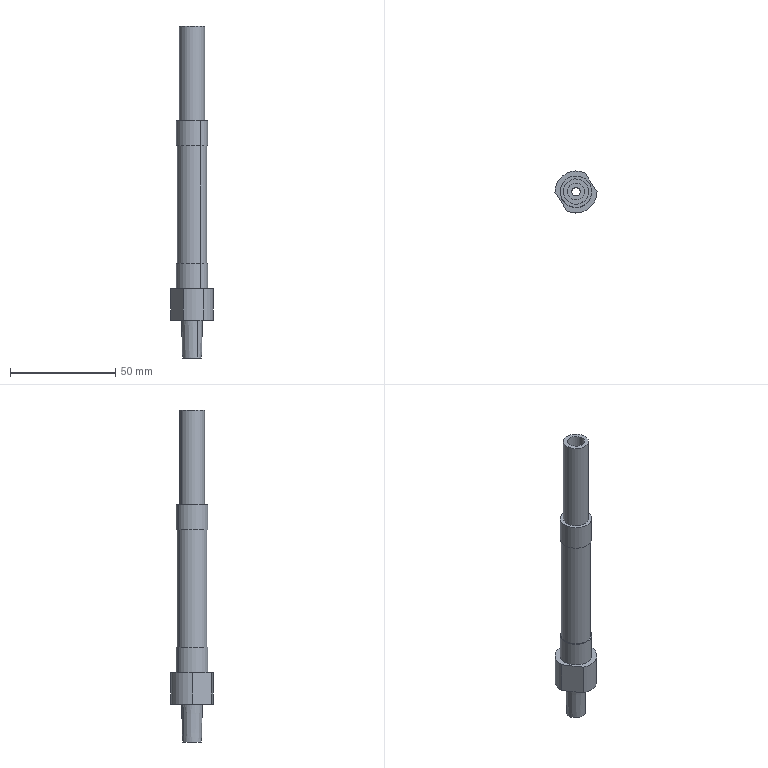Component | SolidWorks | Axis-2 | 1 solid | 27 faces | box 20 x 20 x 158 mm | volume 19937 mm3 | cylinder 15 | plane 10 | cone 2 | commonest cylinder face diameters 15 x4 20 x3 4 x2 8 x2 12 x2 14 x2
build123d program:
from build123d import *

# Parameters (mm, degrees)
SKETCH3_R      = 4
EXTRUDE1_DEPTH = 45
SKETCH4_R      = 2
EXTRUDE2_DEPTH = 159.632
SKETCH5_W      = 1.5
SKETCH5_H      = 15
EXTRUDE3_DEPTH = 10


with BuildPart() as part:
    # Sketch1 → Revolve1 (revolve)
    with BuildSketch(Plane.XY, mode=Mode.PRIVATE) as revolve1_sk:
        Polygon((0, 52.72), (4.5, 52.72), (5, 34.72), (10, 34.72), (10, 19.72), (7.5, 19.72), (7.5, 7.72), (7, 7.72), (7, -48.28), (7.5, -48.28), (7.5, -60.28), (6, -60.28), (6, -105.28), (0, -105.28), align=None)
    revolve(revolve1_sk.sketch.rotate(Axis((0, 0, 0), (0, 1, 0)), 90), axis=Axis((0, 0, 0), (0, 1, 0)))

    # Sketch3 → Extrude1 (cut)
    with BuildSketch(Plane.XZ.offset(105.28)):
        with Locations(Location((0, 0, 0), (0, 0, 270))):
            Circle(SKETCH3_R)
    extrude(amount=-EXTRUDE1_DEPTH, mode=Mode.SUBTRACT)

    # Sketch4 → Extrude2 (cut, through all)
    with BuildSketch(Plane(origin=(0, 52.72, 0), x_dir=(1, 0, 0), z_dir=(0, 1, 0))):
        with Locations(Location((0, 0, 0), (0, 0, 270))):
            Circle(SKETCH4_R)
    extrude(amount=-EXTRUDE2_DEPTH, mode=Mode.SUBTRACT)

    # Sketch5 → Extrude3 (cut, symmetric)
    with BuildSketch(Plane.XY):
        with Locations((9.25, 27.22)):
            Rectangle(SKETCH5_W, SKETCH5_H)
        with Locations((-9.25, 27.22)):
            Rectangle(SKETCH5_W, SKETCH5_H)
    extrude(amount=EXTRUDE3_DEPTH, both=True, mode=Mode.SUBTRACT)


solid = part.part

# Placed as in the assembly
solid = solid.moved(Location((-110.944, 573.983, 177.508), (-90, -33.719, 0)))
STEP:
#1=COLOUR_RGB('',0.7922,0.8196,0.9333);
#2=FILL_AREA_STYLE_COLOUR('',#1);
#3=FILL_AREA_STYLE('',(#2));
#4=SURFACE_STYLE_FILL_AREA(#3);
#5=SURFACE_SIDE_STYLE('',(#4));
#6=SURFACE_STYLE_USAGE(.BOTH.,#5);
#7=PRESENTATION_STYLE_ASSIGNMENT((#6));
#8=CARTESIAN_POINT('',(-4.412,22.663,9.362));
#9=VERTEX_POINT('',#8);
#10=CARTESIAN_POINT('',(-4.324,22.532,9.362));
#11=VERTEX_POINT('',#10);
#12=CARTESIAN_POINT('',(-4.368,22.598,9.362));
#13=DIRECTION('',(0.,0.,1.));
#14=DIRECTION('',(0.5551,-0.8318,0.));
#15=AXIS2_PLACEMENT_3D('',#12,#13,#14);
#16=CIRCLE('',#15,0.07874);
#17=EDGE_CURVE('',#9,#11,#16,.T.);
#18=ORIENTED_EDGE('',*,*,#17,.T.);
#19=CARTESIAN_POINT('',(-4.324,22.532,4.913));
#20=VERTEX_POINT('',#19);
#21=CARTESIAN_POINT('',(-4.324,22.532,11.133));
#22=DIRECTION('',(0.,0.,-1.));
#23=VECTOR('',#22,39.37);
#24=LINE('',#21,#23);
#25=EDGE_CURVE('',#11,#20,#24,.T.);
#26=ORIENTED_EDGE('',*,*,#25,.T.);
#27=CARTESIAN_POINT('',(-4.412,22.663,4.913));
#28=VERTEX_POINT('',#27);
#29=CARTESIAN_POINT('',(-4.368,22.598,4.913));
#30=DIRECTION('',(0.,0.,-1.));
#31=DIRECTION('',(-0.5551,0.8318,0.));
#32=AXIS2_PLACEMENT_3D('',#29,#30,#31);
#33=CIRCLE('',#32,0.07874);
#34=EDGE_CURVE('',#20,#28,#33,.T.);
#35=ORIENTED_EDGE('',*,*,#34,.T.);
#36=CARTESIAN_POINT('',(-4.412,22.663,11.133));
#37=DIRECTION('',(0.,0.,-1.));
#38=VECTOR('',#37,39.37);
#39=LINE('',#36,#38);
#40=EDGE_CURVE('',#9,#28,#39,.T.);
#41=ORIENTED_EDGE('',*,*,#40,.F.);
#42=EDGE_LOOP('',(#18,#26,#35,#41));
#43=FACE_OUTER_BOUND('',#42,.T.);
#44=CARTESIAN_POINT('',(-4.368,22.598,11.133));
#45=DIRECTION('',(0.,0.,-1.));
#46=DIRECTION('',(-0.5551,0.8318,0.));
#47=AXIS2_PLACEMENT_3D('',#44,#45,#46);
#48=CYLINDRICAL_SURFACE('',#47,0.07874);
#49=ADVANCED_FACE('',(#43),#48,.F.);
#50=CARTESIAN_POINT('',(-4.28,22.467,9.362));
#51=VERTEX_POINT('',#50);
#52=CARTESIAN_POINT('',(-4.455,22.729,9.362));
#53=VERTEX_POINT('',#52);
#54=CARTESIAN_POINT('',(-4.368,22.598,9.362));
#55=DIRECTION('',(0.,0.,-1.));
#56=DIRECTION('',(0.5551,-0.8318,0.));
#57=AXIS2_PLACEMENT_3D('',#54,#55,#56);
#58=CIRCLE('',#57,0.1575);
#59=EDGE_CURVE('',#51,#53,#58,.T.);
#60=ORIENTED_EDGE('',*,*,#59,.T.);
#61=CARTESIAN_POINT('',(-4.455,22.729,11.133));
#62=VERTEX_POINT('',#61);
#63=CARTESIAN_POINT('',(-4.455,22.729,8.916));
#64=DIRECTION('',(0.,0.,1.));
#65=VECTOR('',#64,39.37);
#66=LINE('',#63,#65);
#67=EDGE_CURVE('',#53,#62,#66,.T.);
#68=ORIENTED_EDGE('',*,*,#67,.T.);
#69=CARTESIAN_POINT('',(-4.28,22.467,11.133));
#70=VERTEX_POINT('',#69);
#71=CARTESIAN_POINT('',(-4.368,22.598,11.133));
#72=DIRECTION('',(0.,0.,1.));
#73=DIRECTION('',(0.5551,-0.8318,0.));
#74=AXIS2_PLACEMENT_3D('',#71,#72,#73);
#75=CIRCLE('',#74,0.1575);
#76=EDGE_CURVE('',#62,#70,#75,.T.);
#77=ORIENTED_EDGE('',*,*,#76,.T.);
#78=CARTESIAN_POINT('',(-4.28,22.467,8.916));
#79=DIRECTION('',(0.,0.,1.));
#80=VECTOR('',#79,39.37);
#81=LINE('',#78,#80);
#82=EDGE_CURVE('',#51,#70,#81,.T.);
#83=ORIENTED_EDGE('',*,*,#82,.F.);
#84=EDGE_LOOP('',(#60,#68,#77,#83));
#85=FACE_OUTER_BOUND('',#84,.T.);
#86=CARTESIAN_POINT('',(-4.368,22.598,8.916));
#87=DIRECTION('',(0.,0.,1.));
#88=DIRECTION('',(0.5551,-0.8318,0.));
#89=AXIS2_PLACEMENT_3D('',#86,#87,#88);
#90=CYLINDRICAL_SURFACE('',#89,0.1575);
#91=ADVANCED_FACE('',(#85),#90,.F.);
#92=CARTESIAN_POINT('',(-4.237,22.401,9.362));
#93=VERTEX_POINT('',#92);
#94=CARTESIAN_POINT('',(-4.499,22.794,9.362));
#95=VERTEX_POINT('',#94);
#96=CARTESIAN_POINT('',(-4.368,22.598,9.362));
#97=DIRECTION('',(0.,0.,1.));
#98=DIRECTION('',(0.5551,-0.8318,0.));
#99=AXIS2_PLACEMENT_3D('',#96,#97,#98);
#100=CIRCLE('',#99,0.2362);
#101=EDGE_CURVE('',#93,#95,#100,.T.);
#102=ORIENTED_EDGE('',*,*,#101,.T.);
#103=CARTESIAN_POINT('',(-4.499,22.794,11.133));
#104=VERTEX_POINT('',#103);
#105=CARTESIAN_POINT('',(-4.499,22.794,6.989));
#106=DIRECTION('',(0.,0.,1.));
#107=VECTOR('',#106,39.37);
#108=LINE('',#105,#107);
#109=EDGE_CURVE('',#95,#104,#108,.T.);
#110=ORIENTED_EDGE('',*,*,#109,.T.);
#111=CARTESIAN_POINT('',(-4.237,22.401,11.133));
#112=VERTEX_POINT('',#111);
#113=CARTESIAN_POINT('',(-4.368,22.598,11.133));
#114=DIRECTION('',(0.,0.,1.));
#115=DIRECTION('',(0.5551,-0.8318,0.));
#116=AXIS2_PLACEMENT_3D('',#113,#114,#115);
#117=CIRCLE('',#116,0.2362);
#118=EDGE_CURVE('',#112,#104,#117,.T.);
#119=ORIENTED_EDGE('',*,*,#118,.F.);
#120=CARTESIAN_POINT('',(-4.237,22.401,6.989));
#121=DIRECTION('',(0.,0.,1.));
#122=VECTOR('',#121,39.37);
#123=LINE('',#120,#122);
#124=EDGE_CURVE('',#93,#112,#123,.T.);
#125=ORIENTED_EDGE('',*,*,#124,.F.);
#126=EDGE_LOOP('',(#102,#110,#119,#125));
#127=FACE_OUTER_BOUND('',#126,.T.);
#128=CARTESIAN_POINT('',(-4.368,22.598,6.989));
#129=DIRECTION('',(0.,0.,1.));
#130=DIRECTION('',(0.5551,-0.8318,0.));
#131=AXIS2_PLACEMENT_3D('',#128,#129,#130);
#132=CYLINDRICAL_SURFACE('',#131,0.2362);
#133=ADVANCED_FACE('',(#127),#132,.T.);
#134=CARTESIAN_POINT('',(-4.204,22.352,8.889));
#135=VERTEX_POINT('',#134);
#136=CARTESIAN_POINT('',(-4.532,22.843,8.889));
#137=VERTEX_POINT('',#136);
#138=CARTESIAN_POINT('',(-4.368,22.598,8.889));
#139=DIRECTION('',(0.,0.,1.));
#140=DIRECTION('',(0.5551,-0.8318,0.));
#141=AXIS2_PLACEMENT_3D('',#138,#139,#140);
#142=CIRCLE('',#141,0.2953);
#143=EDGE_CURVE('',#135,#137,#142,.T.);
#144=ORIENTED_EDGE('',*,*,#143,.T.);
#145=CARTESIAN_POINT('',(-4.532,22.843,9.362));
#146=VERTEX_POINT('',#145);
#147=CARTESIAN_POINT('',(-4.532,22.843,6.989));
#148=DIRECTION('',(0.,0.,1.));
#149=VECTOR('',#148,39.37);
#150=LINE('',#147,#149);
#151=EDGE_CURVE('',#137,#146,#150,.T.);
#152=ORIENTED_EDGE('',*,*,#151,.T.);
#153=CARTESIAN_POINT('',(-4.204,22.352,9.362));
#154=VERTEX_POINT('',#153);
#155=CARTESIAN_POINT('',(-4.368,22.598,9.362));
#156=DIRECTION('',(0.,0.,1.));
#157=DIRECTION('',(0.5551,-0.8318,0.));
#158=AXIS2_PLACEMENT_3D('',#155,#156,#157);
#159=CIRCLE('',#158,0.2953);
#160=EDGE_CURVE('',#154,#146,#159,.T.);
#161=ORIENTED_EDGE('',*,*,#160,.F.);
#162=CARTESIAN_POINT('',(-4.204,22.352,6.989));
#163=DIRECTION('',(0.,0.,1.));
#164=VECTOR('',#163,39.37);
#165=LINE('',#162,#164);
#166=EDGE_CURVE('',#135,#154,#165,.T.);
#167=ORIENTED_EDGE('',*,*,#166,.F.);
#168=EDGE_LOOP('',(#144,#152,#161,#167));
#169=FACE_OUTER_BOUND('',#168,.T.);
#170=CARTESIAN_POINT('',(-4.368,22.598,6.989));
#171=DIRECTION('',(0.,0.,1.));
#172=DIRECTION('',(0.5551,-0.8318,0.));
#173=AXIS2_PLACEMENT_3D('',#170,#171,#172);
#174=CYLINDRICAL_SURFACE('',#173,0.2953);
#175=ADVANCED_FACE('',(#169),#174,.T.);
#176=CARTESIAN_POINT('',(-4.215,22.369,6.685));
#177=VERTEX_POINT('',#176);
#178=CARTESIAN_POINT('',(-4.521,22.827,6.685));
#179=VERTEX_POINT('',#178);
#180=CARTESIAN_POINT('',(-4.368,22.598,6.685));
#181=DIRECTION('',(0.,0.,1.));
#182=DIRECTION('',(0.5551,-0.8318,0.));
#183=AXIS2_PLACEMENT_3D('',#180,#181,#182);
#184=CIRCLE('',#183,0.2756);
#185=EDGE_CURVE('',#177,#179,#184,.T.);
#186=ORIENTED_EDGE('',*,*,#185,.T.);
#187=CARTESIAN_POINT('',(-4.521,22.827,8.889));
#188=VERTEX_POINT('',#187);
#189=CARTESIAN_POINT('',(-4.521,22.827,6.989));
#190=DIRECTION('',(0.,0.,1.));
#191=VECTOR('',#190,39.37);
#192=LINE('',#189,#191);
#193=EDGE_CURVE('',#179,#188,#192,.T.);
#194=ORIENTED_EDGE('',*,*,#193,.T.);
#195=CARTESIAN_POINT('',(-4.215,22.369,8.889));
#196=VERTEX_POINT('',#195);
#197=CARTESIAN_POINT('',(-4.368,22.598,8.889));
#198=DIRECTION('',(0.,0.,1.));
#199=DIRECTION('',(0.5551,-0.8318,0.));
#200=AXIS2_PLACEMENT_3D('',#197,#198,#199);
#201=CIRCLE('',#200,0.2756);
#202=EDGE_CURVE('',#196,#188,#201,.T.);
#203=ORIENTED_EDGE('',*,*,#202,.F.);
#204=CARTESIAN_POINT('',(-4.215,22.369,6.989));
#205=DIRECTION('',(0.,0.,1.));
#206=VECTOR('',#205,39.37);
#207=LINE('',#204,#206);
#208=EDGE_CURVE('',#177,#196,#207,.T.);
#209=ORIENTED_EDGE('',*,*,#208,.F.);
#210=EDGE_LOOP('',(#186,#194,#203,#209));
#211=FACE_OUTER_BOUND('',#210,.T.);
#212=CARTESIAN_POINT('',(-4.368,22.598,6.989));
#213=DIRECTION('',(0.,0.,1.));
#214=DIRECTION('',(0.5551,-0.8318,0.));
#215=AXIS2_PLACEMENT_3D('',#212,#213,#214);
#216=CYLINDRICAL_SURFACE('',#215,0.2756);
#217=ADVANCED_FACE('',(#211),#216,.T.);
#218=CARTESIAN_POINT('',(-4.204,22.352,6.212));
#219=VERTEX_POINT('',#218);
#220=CARTESIAN_POINT('',(-4.532,22.843,6.212));
#221=VERTEX_POINT('',#220);
#222=CARTESIAN_POINT('',(-4.368,22.598,6.212));
#223=DIRECTION('',(0.,0.,1.));
#224=DIRECTION('',(0.5551,-0.8318,0.));
#225=AXIS2_PLACEMENT_3D('',#222,#223,#224);
#226=CIRCLE('',#225,0.2953);
#227=EDGE_CURVE('',#219,#221,#226,.T.);
#228=ORIENTED_EDGE('',*,*,#227,.T.);
#229=CARTESIAN_POINT('',(-4.532,22.843,6.685));
#230=VERTEX_POINT('',#229);
#231=CARTESIAN_POINT('',(-4.532,22.843,6.989));
#232=DIRECTION('',(0.,0.,1.));
#233=VECTOR('',#232,39.37);
#234=LINE('',#231,#233);
#235=EDGE_CURVE('',#221,#230,#234,.T.);
#236=ORIENTED_EDGE('',*,*,#235,.T.);
#237=CARTESIAN_POINT('',(-4.204,22.352,6.685));
#238=VERTEX_POINT('',#237);
#239=CARTESIAN_POINT('',(-4.368,22.598,6.685));
#240=DIRECTION('',(0.,0.,1.));
#241=DIRECTION('',(0.5551,-0.8318,0.));
#242=AXIS2_PLACEMENT_3D('',#239,#240,#241);
#243=CIRCLE('',#242,0.2953);
#244=EDGE_CURVE('',#238,#230,#243,.T.);
#245=ORIENTED_EDGE('',*,*,#244,.F.);
#246=CARTESIAN_POINT('',(-4.204,22.352,6.989));
#247=DIRECTION('',(0.,0.,1.));
#248=VECTOR('',#247,39.37);
#249=LINE('',#246,#248);
#250=EDGE_CURVE('',#219,#238,#249,.T.);
#251=ORIENTED_EDGE('',*,*,#250,.F.);
#252=EDGE_LOOP('',(#228,#236,#245,#251));
#253=FACE_OUTER_BOUND('',#252,.T.);
#254=CARTESIAN_POINT('',(-4.368,22.598,6.989));
#255=DIRECTION('',(0.,0.,1.));
#256=DIRECTION('',(0.5551,-0.8318,0.));
#257=AXIS2_PLACEMENT_3D('',#254,#255,#256);
#258=CYLINDRICAL_SURFACE('',#257,0.2953);
#259=ADVANCED_FACE('',(#253),#258,.T.);
#260=CARTESIAN_POINT('',(-4.531,22.239,5.622));
#261=VERTEX_POINT('',#260);
#262=CARTESIAN_POINT('',(-4.149,22.27,5.622));
#263=VERTEX_POINT('',#262);
#264=CARTESIAN_POINT('',(-4.368,22.598,5.622));
#265=DIRECTION('',(0.,0.,1.));
#266=DIRECTION('',(0.5551,-0.8318,0.));
#267=AXIS2_PLACEMENT_3D('',#264,#265,#266);
#268=CIRCLE('',#267,0.3937);
#269=EDGE_CURVE('',#261,#263,#268,.T.);
#270=ORIENTED_EDGE('',*,*,#269,.T.);
#271=CARTESIAN_POINT('',(-4.149,22.27,6.212));
#272=VERTEX_POINT('',#271);
#273=CARTESIAN_POINT('',(-4.149,22.27,6.989));
#274=DIRECTION('',(0.,0.,1.));
#275=VECTOR('',#274,39.37);
#276=LINE('',#273,#275);
#277=EDGE_CURVE('',#263,#272,#276,.T.);
#278=ORIENTED_EDGE('',*,*,#277,.T.);
#279=CARTESIAN_POINT('',(-4.531,22.239,6.212));
#280=VERTEX_POINT('',#279);
#281=CARTESIAN_POINT('',(-4.368,22.598,6.212));
#282=DIRECTION('',(0.,0.,1.));
#283=DIRECTION('',(0.5551,-0.8318,0.));
#284=AXIS2_PLACEMENT_3D('',#281,#282,#283);
#285=CIRCLE('',#284,0.3937);
#286=EDGE_CURVE('',#280,#272,#285,.T.);
#287=ORIENTED_EDGE('',*,*,#286,.F.);
#288=CARTESIAN_POINT('',(-4.531,22.239,6.989));
#289=DIRECTION('',(0.,0.,1.));
#290=VECTOR('',#289,39.37);
#291=LINE('',#288,#290);
#292=EDGE_CURVE('',#261,#280,#291,.T.);
#293=ORIENTED_EDGE('',*,*,#292,.F.);
#294=EDGE_LOOP('',(#270,#278,#287,#293));
#295=FACE_OUTER_BOUND('',#294,.T.);
#296=CARTESIAN_POINT('',(-4.368,22.598,6.989));
#297=DIRECTION('',(0.,0.,1.));
#298=DIRECTION('',(0.5551,-0.8318,0.));
#299=AXIS2_PLACEMENT_3D('',#296,#297,#298);
#300=CYLINDRICAL_SURFACE('',#299,0.3937);
#301=ADVANCED_FACE('',(#295),#300,.T.);
#302=CARTESIAN_POINT('',(-4.27,22.45,4.913));
#303=VERTEX_POINT('',#302);
#304=CARTESIAN_POINT('',(-4.466,22.745,4.913));
#305=VERTEX_POINT('',#304);
#306=CARTESIAN_POINT('',(-4.368,22.598,4.913));
#307=DIRECTION('',(0.,0.,1.));
#308=DIRECTION('',(0.5551,-0.8318,0.));
#309=AXIS2_PLACEMENT_3D('',#306,#307,#308);
#310=CIRCLE('',#309,0.1772);
#311=EDGE_CURVE('',#303,#305,#310,.T.);
#312=ORIENTED_EDGE('',*,*,#311,.T.);
#313=CARTESIAN_POINT('',(-4.477,22.762,5.622));
#314=VERTEX_POINT('',#313);
#315=CARTESIAN_POINT('',(-4.477,22.762,5.622));
#316=DIRECTION('',(-0.01541,0.0231,0.9996));
#317=VECTOR('',#316,39.37);
#318=LINE('',#315,#317);
#319=EDGE_CURVE('',#305,#314,#318,.T.);
#320=ORIENTED_EDGE('',*,*,#319,.T.);
#321=CARTESIAN_POINT('',(-4.259,22.434,5.622));
#322=VERTEX_POINT('',#321);
#323=CARTESIAN_POINT('',(-4.368,22.598,5.622));
#324=DIRECTION('',(0.,0.,1.));
#325=DIRECTION('',(0.5551,-0.8318,0.));
#326=AXIS2_PLACEMENT_3D('',#323,#324,#325);
#327=CIRCLE('',#326,0.1969);
#328=EDGE_CURVE('',#322,#314,#327,.T.);
#329=ORIENTED_EDGE('',*,*,#328,.F.);
#330=CARTESIAN_POINT('',(-4.259,22.434,5.622));
#331=DIRECTION('',(0.01541,-0.0231,0.9996));
#332=VECTOR('',#331,39.37);
#333=LINE('',#330,#332);
#334=EDGE_CURVE('',#303,#322,#333,.T.);
#335=ORIENTED_EDGE('',*,*,#334,.F.);
#336=EDGE_LOOP('',(#312,#320,#329,#335));
#337=FACE_OUTER_BOUND('',#336,.T.);
#338=CARTESIAN_POINT('',(-4.368,22.598,5.622));
#339=DIRECTION('',(0.,0.,1.));
#340=DIRECTION('',(0.5551,-0.8318,0.));
#341=AXIS2_PLACEMENT_3D('',#338,#339,#340);
#342=CONICAL_SURFACE('',#341,0.1969,0.02777);
#343=ADVANCED_FACE('',(#337),#342,.T.);
#344=CARTESIAN_POINT('',(-4.761,22.585,6.212));
#345=VERTEX_POINT('',#344);
#346=CARTESIAN_POINT('',(-4.761,22.585,5.622));
#347=VERTEX_POINT('',#346);
#348=CARTESIAN_POINT('',(-4.761,22.585,6.989));
#349=DIRECTION('',(0.,0.,-1.));
#350=VECTOR('',#349,39.37);
#351=LINE('',#348,#350);
#352=EDGE_CURVE('',#345,#347,#351,.T.);
#353=ORIENTED_EDGE('',*,*,#352,.F.);
#354=CARTESIAN_POINT('',(-4.205,22.956,6.212));
#355=VERTEX_POINT('',#354);
#356=CARTESIAN_POINT('',(-4.368,22.598,6.212));
#357=DIRECTION('',(0.,0.,1.));
#358=DIRECTION('',(0.5551,-0.8318,0.));
#359=AXIS2_PLACEMENT_3D('',#356,#357,#358);
#360=CIRCLE('',#359,0.3937);
#361=EDGE_CURVE('',#355,#345,#360,.T.);
#362=ORIENTED_EDGE('',*,*,#361,.F.);
#363=CARTESIAN_POINT('',(-4.205,22.956,5.622));
#364=VERTEX_POINT('',#363);
#365=CARTESIAN_POINT('',(-4.205,22.956,6.989));
#366=DIRECTION('',(0.,0.,1.));
#367=VECTOR('',#366,39.37);
#368=LINE('',#365,#367);
#369=EDGE_CURVE('',#364,#355,#368,.T.);
#370=ORIENTED_EDGE('',*,*,#369,.F.);
#371=CARTESIAN_POINT('',(-4.368,22.598,5.622));
#372=DIRECTION('',(0.,0.,1.));
#373=DIRECTION('',(0.5551,-0.8318,0.));
#374=AXIS2_PLACEMENT_3D('',#371,#372,#373);
#375=CIRCLE('',#374,0.3937);
#376=EDGE_CURVE('',#364,#347,#375,.T.);
#377=ORIENTED_EDGE('',*,*,#376,.T.);
#378=EDGE_LOOP('',(#353,#362,#370,#377));
#379=FACE_OUTER_BOUND('',#378,.T.);
#380=CARTESIAN_POINT('',(-4.368,22.598,6.989));
#381=DIRECTION('',(0.,0.,1.));
#382=DIRECTION('',(0.5551,-0.8318,0.));
#383=AXIS2_PLACEMENT_3D('',#380,#381,#382);
#384=CYLINDRICAL_SURFACE('',#383,0.3937);
#385=ADVANCED_FACE('',(#379),#384,.T.);
#386=CARTESIAN_POINT('',(-4.368,22.598,4.913));
#387=DIRECTION('',(0.,0.,-1.));
#388=DIRECTION('',(-0.5551,0.8318,0.));
#389=AXIS2_PLACEMENT_3D('',#386,#387,#388);
#390=CIRCLE('',#389,0.07874);
#391=EDGE_CURVE('',#28,#20,#390,.T.);
#392=ORIENTED_EDGE('',*,*,#391,.F.);
#393=ORIENTED_EDGE('',*,*,#34,.F.);
#394=EDGE_LOOP('',(#392,#393));
#395=FACE_BOUND('',#394,.T.);
#396=ORIENTED_EDGE('',*,*,#311,.F.);
#397=CARTESIAN_POINT('',(-4.368,22.598,4.913));
#398=DIRECTION('',(0.,0.,1.));
#399=DIRECTION('',(0.5551,-0.8318,0.));
#400=AXIS2_PLACEMENT_3D('',#397,#398,#399);
#401=CIRCLE('',#400,0.1772);
#402=EDGE_CURVE('',#305,#303,#401,.T.);
#403=ORIENTED_EDGE('',*,*,#402,.F.);
#404=EDGE_LOOP('',(#396,#403));
#405=FACE_OUTER_BOUND('',#404,.T.);
#406=CARTESIAN_POINT('',(-4.368,22.598,4.913));
#407=DIRECTION('',(0.,0.,-1.));
#408=DIRECTION('',(-0.5551,0.8318,0.));
#409=AXIS2_PLACEMENT_3D('',#406,#407,#408);
#410=PLANE('',#409);
#411=ADVANCED_FACE('',(#395,#405),#410,.T.);
#412=ORIENTED_EDGE('',*,*,#319,.F.);
#413=ORIENTED_EDGE('',*,*,#402,.T.);
#414=ORIENTED_EDGE('',*,*,#334,.T.);
#415=CARTESIAN_POINT('',(-4.368,22.598,5.622));
#416=DIRECTION('',(0.,0.,1.));
#417=DIRECTION('',(0.5551,-0.8318,0.));
#418=AXIS2_PLACEMENT_3D('',#415,#416,#417);
#419=CIRCLE('',#418,0.1969);
#420=EDGE_CURVE('',#314,#322,#419,.T.);
#421=ORIENTED_EDGE('',*,*,#420,.F.);
#422=EDGE_LOOP('',(#412,#413,#414,#421));
#423=FACE_OUTER_BOUND('',#422,.T.);
#424=CARTESIAN_POINT('',(-4.368,22.598,5.622));
#425=DIRECTION('',(0.,0.,1.));
#426=DIRECTION('',(0.5551,-0.8318,0.));
#427=AXIS2_PLACEMENT_3D('',#424,#425,#426);
#428=CONICAL_SURFACE('',#427,0.1969,0.02777);
#429=ADVANCED_FACE('',(#423),#428,.T.);
#430=CARTESIAN_POINT('',(-4.428,22.085,5.622));
#431=DIRECTION('',(-0.5551,0.8318,0.));
#432=VECTOR('',#431,39.37);
#433=LINE('',#430,#432);
#434=EDGE_CURVE('',#261,#347,#433,.T.);
#435=ORIENTED_EDGE('',*,*,#434,.T.);
#436=ORIENTED_EDGE('',*,*,#376,.F.);
#437=CARTESIAN_POINT('',(-3.974,22.611,5.622));
#438=VERTEX_POINT('',#437);
#439=CARTESIAN_POINT('',(-3.871,22.456,5.622));
#440=DIRECTION('',(-0.5551,0.8318,0.));
#441=VECTOR('',#440,39.37);
#442=LINE('',#439,#441);
#443=EDGE_CURVE('',#438,#364,#442,.T.);
#444=ORIENTED_EDGE('',*,*,#443,.F.);
#445=CARTESIAN_POINT('',(-4.368,22.598,5.622));
#446=DIRECTION('',(0.,0.,1.));
#447=DIRECTION('',(0.5551,-0.8318,0.));
#448=AXIS2_PLACEMENT_3D('',#445,#446,#447);
#449=CIRCLE('',#448,0.3937);
#450=EDGE_CURVE('',#263,#438,#449,.T.);
#451=ORIENTED_EDGE('',*,*,#450,.F.);
#452=ORIENTED_EDGE('',*,*,#269,.F.);
#453=EDGE_LOOP('',(#435,#436,#444,#451,#452));
#454=FACE_OUTER_BOUND('',#453,.T.);
#455=ORIENTED_EDGE('',*,*,#328,.T.);
#456=ORIENTED_EDGE('',*,*,#420,.T.);
#457=EDGE_LOOP('',(#455,#456));
#458=FACE_BOUND('',#457,.T.);
#459=CARTESIAN_POINT('',(-4.204,22.707,5.622));
#460=DIRECTION('',(0.,0.,-1.));
#461=DIRECTION('',(-0.5551,0.8318,0.));
#462=AXIS2_PLACEMENT_3D('',#459,#460,#461);
#463=PLANE('',#462);
#464=ADVANCED_FACE('',(#454,#458),#463,.T.);
#465=ORIENTED_EDGE('',*,*,#277,.F.);
#466=ORIENTED_EDGE('',*,*,#450,.T.);
#467=CARTESIAN_POINT('',(-3.974,22.611,6.212));
#468=VERTEX_POINT('',#467);
#469=CARTESIAN_POINT('',(-3.974,22.611,6.989));
#470=DIRECTION('',(0.,0.,-1.));
#471=VECTOR('',#470,39.37);
#472=LINE('',#469,#471);
#473=EDGE_CURVE('',#468,#438,#472,.T.);
#474=ORIENTED_EDGE('',*,*,#473,.F.);
#475=CARTESIAN_POINT('',(-4.368,22.598,6.212));
#476=DIRECTION('',(0.,0.,1.));
#477=DIRECTION('',(0.5551,-0.8318,0.));
#478=AXIS2_PLACEMENT_3D('',#475,#476,#477);
#479=CIRCLE('',#478,0.3937);
#480=EDGE_CURVE('',#272,#468,#479,.T.);
#481=ORIENTED_EDGE('',*,*,#480,.F.);
#482=EDGE_LOOP('',(#465,#466,#474,#481));
#483=FACE_OUTER_BOUND('',#482,.T.);
#484=CARTESIAN_POINT('',(-4.368,22.598,6.989));
#485=DIRECTION('',(0.,0.,1.));
#486=DIRECTION('',(0.5551,-0.8318,0.));
#487=AXIS2_PLACEMENT_3D('',#484,#485,#486);
#488=CYLINDRICAL_SURFACE('',#487,0.3937);
#489=ADVANCED_FACE('',(#483),#488,.T.);
#490=CARTESIAN_POINT('',(-4.646,22.412,6.212));
#491=DIRECTION('',(-0.5551,0.8318,0.));
#492=VECTOR('',#491,39.37);
#493=LINE('',#490,#492);
#494=EDGE_CURVE('',#280,#345,#493,.T.);
#495=ORIENTED_EDGE('',*,*,#494,.F.);
#496=ORIENTED_EDGE('',*,*,#286,.T.);
#497=ORIENTED_EDGE('',*,*,#480,.T.);
#498=CARTESIAN_POINT('',(-4.09,22.784,6.212));
#499=DIRECTION('',(0.5551,-0.8318,0.));
#500=VECTOR('',#499,39.37);
#501=LINE('',#498,#500);
#502=EDGE_CURVE('',#355,#468,#501,.T.);
#503=ORIENTED_EDGE('',*,*,#502,.F.);
#504=ORIENTED_EDGE('',*,*,#361,.T.);
#505=EDGE_LOOP('',(#495,#496,#497,#503,#504));
#506=FACE_OUTER_BOUND('',#505,.T.);
#507=ORIENTED_EDGE('',*,*,#227,.F.);
#508=CARTESIAN_POINT('',(-4.368,22.598,6.212));
#509=DIRECTION('',(0.,0.,1.));
#510=DIRECTION('',(0.5551,-0.8318,0.));
#511=AXIS2_PLACEMENT_3D('',#508,#509,#510);
#512=CIRCLE('',#511,0.2953);
#513=EDGE_CURVE('',#221,#219,#512,.T.);
#514=ORIENTED_EDGE('',*,*,#513,.F.);
#515=EDGE_LOOP('',(#507,#514));
#516=FACE_BOUND('',#515,.T.);
#517=CARTESIAN_POINT('',(-4.04,22.816,6.212));
#518=DIRECTION('',(0.,0.,1.));
#519=DIRECTION('',(0.5551,-0.8318,0.));
#520=AXIS2_PLACEMENT_3D('',#517,#518,#519);
#521=PLANE('',#520);
#522=ADVANCED_FACE('',(#506,#516),#521,.T.);
#523=ORIENTED_EDGE('',*,*,#235,.F.);
#524=ORIENTED_EDGE('',*,*,#513,.T.);
#525=ORIENTED_EDGE('',*,*,#250,.T.);
#526=CARTESIAN_POINT('',(-4.368,22.598,6.685));
#527=DIRECTION('',(0.,0.,1.));
#528=DIRECTION('',(0.5551,-0.8318,0.));
#529=AXIS2_PLACEMENT_3D('',#526,#527,#528);
#530=CIRCLE('',#529,0.2953);
#531=EDGE_CURVE('',#230,#238,#530,.T.);
#532=ORIENTED_EDGE('',*,*,#531,.F.);
#533=EDGE_LOOP('',(#523,#524,#525,#532));
#534=FACE_OUTER_BOUND('',#533,.T.);
#535=CARTESIAN_POINT('',(-4.368,22.598,6.989));
#536=DIRECTION('',(0.,0.,1.));
#537=DIRECTION('',(0.5551,-0.8318,0.));
#538=AXIS2_PLACEMENT_3D('',#535,#536,#537);
#539=CYLINDRICAL_SURFACE('',#538,0.2953);
#540=ADVANCED_FACE('',(#534),#539,.T.);
#541=ORIENTED_EDGE('',*,*,#244,.T.);
#542=ORIENTED_EDGE('',*,*,#531,.T.);
#543=EDGE_LOOP('',(#541,#542));
#544=FACE_OUTER_BOUND('',#543,.T.);
#545=ORIENTED_EDGE('',*,*,#185,.F.);
#546=CARTESIAN_POINT('',(-4.368,22.598,6.685));
#547=DIRECTION('',(0.,0.,1.));
#548=DIRECTION('',(0.5551,-0.8318,0.));
#549=AXIS2_PLACEMENT_3D('',#546,#547,#548);
#550=CIRCLE('',#549,0.2756);
#551=EDGE_CURVE('',#179,#177,#550,.T.);
#552=ORIENTED_EDGE('',*,*,#551,.F.);
#553=EDGE_LOOP('',(#545,#552));
#554=FACE_BOUND('',#553,.T.);
#555=CARTESIAN_POINT('',(-4.122,22.762,6.685));
#556=DIRECTION('',(0.,0.,1.));
#557=DIRECTION('',(0.5551,-0.8318,0.));
#558=AXIS2_PLACEMENT_3D('',#555,#556,#557);
#559=PLANE('',#558);
#560=ADVANCED_FACE('',(#544,#554),#559,.T.);
#561=ORIENTED_EDGE('',*,*,#193,.F.);
#562=ORIENTED_EDGE('',*,*,#551,.T.);
#563=ORIENTED_EDGE('',*,*,#208,.T.);
#564=CARTESIAN_POINT('',(-4.368,22.598,8.889));
#565=DIRECTION('',(0.,0.,1.));
#566=DIRECTION('',(0.5551,-0.8318,0.));
#567=AXIS2_PLACEMENT_3D('',#564,#565,#566);
#568=CIRCLE('',#567,0.2756);
#569=EDGE_CURVE('',#188,#196,#568,.T.);
#570=ORIENTED_EDGE('',*,*,#569,.F.);
#571=EDGE_LOOP('',(#561,#562,#563,#570));
#572=FACE_OUTER_BOUND('',#571,.T.);
#573=CARTESIAN_POINT('',(-4.368,22.598,6.989));
#574=DIRECTION('',(0.,0.,1.));
#575=DIRECTION('',(0.5551,-0.8318,0.));
#576=AXIS2_PLACEMENT_3D('',#573,#574,#575);
#577=CYLINDRICAL_SURFACE('',#576,0.2756);
#578=ADVANCED_FACE('',(#572),#577,.T.);
#579=ORIENTED_EDGE('',*,*,#202,.T.);
#580=ORIENTED_EDGE('',*,*,#569,.T.);
#581=EDGE_LOOP('',(#579,#580));
#582=FACE_BOUND('',#581,.T.);
#583=ORIENTED_EDGE('',*,*,#143,.F.);
#584=CARTESIAN_POINT('',(-4.368,22.598,8.889));
#585=DIRECTION('',(0.,0.,1.));
#586=DIRECTION('',(0.5551,-0.8318,0.));
#587=AXIS2_PLACEMENT_3D('',#584,#585,#586);
#588=CIRCLE('',#587,0.2953);
#589=EDGE_CURVE('',#137,#135,#588,.T.);
#590=ORIENTED_EDGE('',*,*,#589,.F.);
#591=EDGE_LOOP('',(#583,#590));
#592=FACE_OUTER_BOUND('',#591,.T.);
#593=CARTESIAN_POINT('',(-4.139,22.751,8.889));
#594=DIRECTION('',(0.,0.,-1.));
#595=DIRECTION('',(-0.5551,0.8318,0.));
#596=AXIS2_PLACEMENT_3D('',#593,#594,#595);
#597=PLANE('',#596);
#598=ADVANCED_FACE('',(#582,#592),#597,.T.);
#599=ORIENTED_EDGE('',*,*,#151,.F.);
#600=ORIENTED_EDGE('',*,*,#589,.T.);
#601=ORIENTED_EDGE('',*,*,#166,.T.);
#602=CARTESIAN_POINT('',(-4.368,22.598,9.362));
#603=DIRECTION('',(0.,0.,1.));
#604=DIRECTION('',(0.5551,-0.8318,0.));
#605=AXIS2_PLACEMENT_3D('',#602,#603,#604);
#606=CIRCLE('',#605,0.2953);
#607=EDGE_CURVE('',#146,#154,#606,.T.);
#608=ORIENTED_EDGE('',*,*,#607,.F.);
#609=EDGE_LOOP('',(#599,#600,#601,#608));
#610=FACE_OUTER_BOUND('',#609,.T.);
#611=CARTESIAN_POINT('',(-4.368,22.598,6.989));
#612=DIRECTION('',(0.,0.,1.));
#613=DIRECTION('',(0.5551,-0.8318,0.));
#614=AXIS2_PLACEMENT_3D('',#611,#612,#613);
#615=CYLINDRICAL_SURFACE('',#614,0.2953);
#616=ADVANCED_FACE('',(#610),#615,.T.);
#617=ORIENTED_EDGE('',*,*,#160,.T.);
#618=ORIENTED_EDGE('',*,*,#607,.T.);
#619=EDGE_LOOP('',(#617,#618));
#620=FACE_OUTER_BOUND('',#619,.T.);
#621=ORIENTED_EDGE('',*,*,#101,.F.);
#622=CARTESIAN_POINT('',(-4.368,22.598,9.362));
#623=DIRECTION('',(0.,0.,1.));
#624=DIRECTION('',(0.5551,-0.8318,0.));
#625=AXIS2_PLACEMENT_3D('',#622,#623,#624);
#626=CIRCLE('',#625,0.2362);
#627=EDGE_CURVE('',#95,#93,#626,.T.);
#628=ORIENTED_EDGE('',*,*,#627,.F.);
#629=EDGE_LOOP('',(#621,#628));
#630=FACE_BOUND('',#629,.T.);
#631=CARTESIAN_POINT('',(-4.122,22.762,9.362));
#632=DIRECTION('',(0.,0.,1.));
#633=DIRECTION('',(0.5551,-0.8318,0.));
#634=AXIS2_PLACEMENT_3D('',#631,#632,#633);
#635=PLANE('',#634);
#636=ADVANCED_FACE('',(#620,#630),#635,.T.);
#637=ORIENTED_EDGE('',*,*,#109,.F.);
#638=ORIENTED_EDGE('',*,*,#627,.T.);
#639=ORIENTED_EDGE('',*,*,#124,.T.);
#640=CARTESIAN_POINT('',(-4.368,22.598,11.133));
#641=DIRECTION('',(0.,0.,1.));
#642=DIRECTION('',(0.5551,-0.8318,0.));
#643=AXIS2_PLACEMENT_3D('',#640,#641,#642);
#644=CIRCLE('',#643,0.2362);
#645=EDGE_CURVE('',#104,#112,#644,.T.);
#646=ORIENTED_EDGE('',*,*,#645,.F.);
#647=EDGE_LOOP('',(#637,#638,#639,#646));
#648=FACE_OUTER_BOUND('',#647,.T.);
#649=CARTESIAN_POINT('',(-4.368,22.598,6.989));
#650=DIRECTION('',(0.,0.,1.));
#651=DIRECTION('',(0.5551,-0.8318,0.));
#652=AXIS2_PLACEMENT_3D('',#649,#650,#651);
#653=CYLINDRICAL_SURFACE('',#652,0.2362);
#654=ADVANCED_FACE('',(#648),#653,.T.);
#655=CARTESIAN_POINT('',(-4.368,22.598,11.133));
#656=DIRECTION('',(0.,0.,1.));
#657=DIRECTION('',(0.5551,-0.8318,0.));
#658=AXIS2_PLACEMENT_3D('',#655,#656,#657);
#659=CIRCLE('',#658,0.1575);
#660=EDGE_CURVE('',#70,#62,#659,.T.);
#661=ORIENTED_EDGE('',*,*,#660,.F.);
#662=ORIENTED_EDGE('',*,*,#76,.F.);
#663=EDGE_LOOP('',(#661,#662));
#664=FACE_BOUND('',#663,.T.);
#665=ORIENTED_EDGE('',*,*,#118,.T.);
#666=ORIENTED_EDGE('',*,*,#645,.T.);
#667=EDGE_LOOP('',(#665,#666));
#668=FACE_OUTER_BOUND('',#667,.T.);
#669=CARTESIAN_POINT('',(-4.171,22.729,11.133));
#670=DIRECTION('',(0.,0.,1.));
#671=DIRECTION('',(0.5551,-0.8318,0.));
#672=AXIS2_PLACEMENT_3D('',#669,#670,#671);
#673=PLANE('',#672);
#674=ADVANCED_FACE('',(#664,#668),#673,.T.);
#675=ORIENTED_EDGE('',*,*,#67,.F.);
#676=CARTESIAN_POINT('',(-4.368,22.598,9.362));
#677=DIRECTION('',(0.,0.,-1.));
#678=DIRECTION('',(0.5551,-0.8318,0.));
#679=AXIS2_PLACEMENT_3D('',#676,#677,#678);
#680=CIRCLE('',#679,0.1575);
#681=EDGE_CURVE('',#53,#51,#680,.T.);
#682=ORIENTED_EDGE('',*,*,#681,.T.);
#683=ORIENTED_EDGE('',*,*,#82,.T.);
#684=ORIENTED_EDGE('',*,*,#660,.T.);
#685=EDGE_LOOP('',(#675,#682,#683,#684));
#686=FACE_OUTER_BOUND('',#685,.T.);
#687=CARTESIAN_POINT('',(-4.368,22.598,8.916));
#688=DIRECTION('',(0.,0.,1.));
#689=DIRECTION('',(0.5551,-0.8318,0.));
#690=AXIS2_PLACEMENT_3D('',#687,#688,#689);
#691=CYLINDRICAL_SURFACE('',#690,0.1575);
#692=ADVANCED_FACE('',(#686),#691,.F.);
#693=ORIENTED_EDGE('',*,*,#17,.F.);
#694=CARTESIAN_POINT('',(-4.368,22.598,9.362));
#695=DIRECTION('',(0.,0.,1.));
#696=DIRECTION('',(0.5551,-0.8318,0.));
#697=AXIS2_PLACEMENT_3D('',#694,#695,#696);
#698=CIRCLE('',#697,0.07874);
#699=EDGE_CURVE('',#11,#9,#698,.T.);
#700=ORIENTED_EDGE('',*,*,#699,.F.);
#701=EDGE_LOOP('',(#693,#700));
#702=FACE_BOUND('',#701,.T.);
#703=ORIENTED_EDGE('',*,*,#59,.F.);
#704=ORIENTED_EDGE('',*,*,#681,.F.);
#705=EDGE_LOOP('',(#703,#704));
#706=FACE_OUTER_BOUND('',#705,.T.);
#707=CARTESIAN_POINT('',(-4.122,22.762,9.362));
#708=DIRECTION('',(0.,0.,1.));
#709=DIRECTION('',(0.5551,-0.8318,0.));
#710=AXIS2_PLACEMENT_3D('',#707,#708,#709);
#711=PLANE('',#710);
#712=ADVANCED_FACE('',(#702,#706),#711,.T.);
#713=ORIENTED_EDGE('',*,*,#25,.F.);
#714=ORIENTED_EDGE('',*,*,#699,.T.);
#715=ORIENTED_EDGE('',*,*,#40,.T.);
#716=ORIENTED_EDGE('',*,*,#391,.T.);
#717=EDGE_LOOP('',(#713,#714,#715,#716));
#718=FACE_OUTER_BOUND('',#717,.T.);
#719=CARTESIAN_POINT('',(-4.368,22.598,11.133));
#720=DIRECTION('',(0.,0.,-1.));
#721=DIRECTION('',(-0.5551,0.8318,0.));
#722=AXIS2_PLACEMENT_3D('',#719,#720,#721);
#723=CYLINDRICAL_SURFACE('',#722,0.07874);
#724=ADVANCED_FACE('',(#718),#723,.F.);
#725=ORIENTED_EDGE('',*,*,#473,.T.);
#726=ORIENTED_EDGE('',*,*,#443,.T.);
#727=ORIENTED_EDGE('',*,*,#369,.T.);
#728=ORIENTED_EDGE('',*,*,#502,.T.);
#729=EDGE_LOOP('',(#725,#726,#727,#728));
#730=FACE_OUTER_BOUND('',#729,.T.);
#731=CARTESIAN_POINT('',(-3.871,22.456,5.622));
#732=DIRECTION('',(-0.8318,-0.5551,0.));
#733=DIRECTION('',(0.,0.,1.));
#734=AXIS2_PLACEMENT_3D('',#731,#732,#733);
#735=PLANE('',#734);
#736=ADVANCED_FACE('',(#730),#735,.F.);
#737=ORIENTED_EDGE('',*,*,#352,.T.);
#738=ORIENTED_EDGE('',*,*,#434,.F.);
#739=ORIENTED_EDGE('',*,*,#292,.T.);
#740=ORIENTED_EDGE('',*,*,#494,.T.);
#741=EDGE_LOOP('',(#737,#738,#739,#740));
#742=FACE_OUTER_BOUND('',#741,.T.);
#743=CARTESIAN_POINT('',(-4.428,22.085,5.622));
#744=DIRECTION('',(0.8318,0.5551,-0.));
#745=DIRECTION('',(-0.,-0.,-1.));
#746=AXIS2_PLACEMENT_3D('',#743,#744,#745);
#747=PLANE('',#746);
#748=ADVANCED_FACE('',(#742),#747,.F.);
#749=CLOSED_SHELL('',(#49,#91,#133,#175,#217,#259,#301,#343,#385,#411,#429,#464,#489,#522,#540,#560,#578,#598,#616,#636,#654,#674,#692,#712,#724,#736,#748));
#750=MANIFOLD_SOLID_BREP('',#749);
#751=STYLED_ITEM('',(#7),#750);
#752=PRESENTATION_LAYER_ASSIGNMENT('','',(#751));
#753=CARTESIAN_POINT('',(0.,0.,0.));
#754=DIRECTION('',(0.,0.,1.));
#755=DIRECTION('',(1.,0.,0.));
#756=AXIS2_PLACEMENT_3D('',#753,#754,#755);
#757=(LENGTH_UNIT()NAMED_UNIT(*)SI_UNIT($,.METRE.));
#758=LENGTH_MEASURE_WITH_UNIT(LENGTH_MEASURE(0.0254),#757);
#759=DIMENSIONAL_EXPONENTS(1.,0.,0.,0.,0.,0.,0.);
#760=(CONVERSION_BASED_UNIT('',#758)LENGTH_UNIT()NAMED_UNIT(#759));
#761=UNCERTAINTY_MEASURE_WITH_UNIT(LENGTH_MEASURE(0.00001),#760,'','');
#762=(NAMED_UNIT(*)PLANE_ANGLE_UNIT()SI_UNIT($,.RADIAN.));
#763=(NAMED_UNIT(*)SI_UNIT($,.STERADIAN.)SOLID_ANGLE_UNIT());
#764=(GEOMETRIC_REPRESENTATION_CONTEXT(3)GLOBAL_UNCERTAINTY_ASSIGNED_CONTEXT((#761))GLOBAL_UNIT_ASSIGNED_CONTEXT((#760,#762,#763))REPRESENTATION_CONTEXT('',''));
#765=ADVANCED_BREP_SHAPE_REPRESENTATION('',(#750,#756),#764);
#766=(LENGTH_UNIT()NAMED_UNIT(*)SI_UNIT($,.METRE.));
#767=LENGTH_MEASURE_WITH_UNIT(LENGTH_MEASURE(0.0254),#766);
#768=DIMENSIONAL_EXPONENTS(1.,0.,0.,0.,0.,0.,0.);
#769=(CONVERSION_BASED_UNIT('',#767)LENGTH_UNIT()NAMED_UNIT(#768));
#770=UNCERTAINTY_MEASURE_WITH_UNIT(LENGTH_MEASURE(0.00001),#769,'','');
#771=(NAMED_UNIT(*)PLANE_ANGLE_UNIT()SI_UNIT($,.RADIAN.));
#772=(NAMED_UNIT(*)SI_UNIT($,.STERADIAN.)SOLID_ANGLE_UNIT());
#773=(GEOMETRIC_REPRESENTATION_CONTEXT(3)GLOBAL_UNCERTAINTY_ASSIGNED_CONTEXT((#770))GLOBAL_UNIT_ASSIGNED_CONTEXT((#769,#771,#772))REPRESENTATION_CONTEXT('',''));
#774=MECHANICAL_DESIGN_GEOMETRIC_PRESENTATION_REPRESENTATION('',(#751),#773);